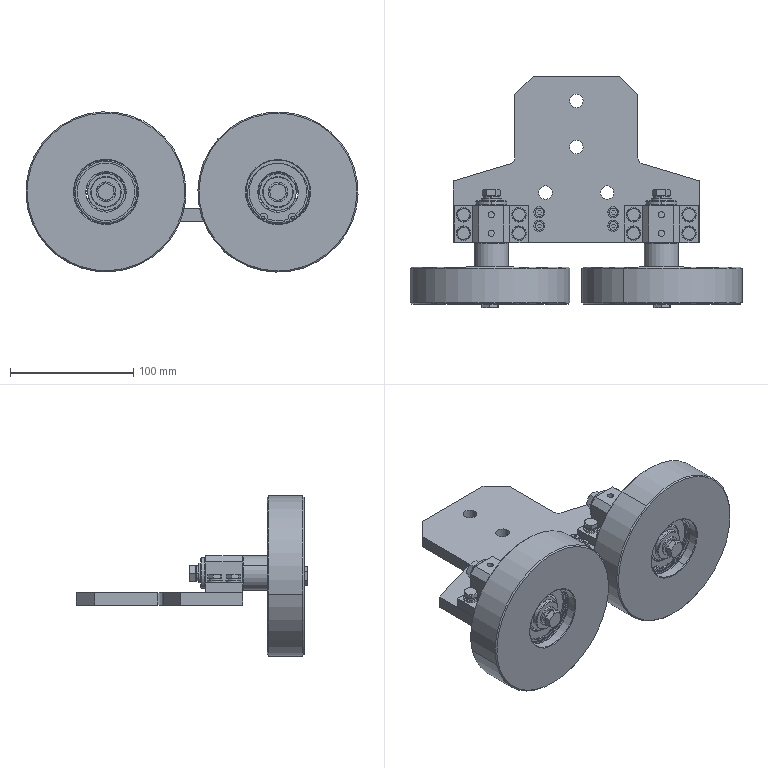Assembly | SolidWorks | mm | 62 component files | 62 solids | 1327 faces | box 269.61 x 188 x 130.18 mm | volume 1018572 mm3 | plane 426 | cylinder 405 | cone 276 | sphere 112 | torus 108 | commonest cylinder face diameters 6 x35 7 x24 6.1 x24 9.282 x24 9 x24 10 x18 4 x16 20 x16
Bill of materials:
Deep Groove Ball Bearing 6304-2RZ | 2 | Alloy Steel | Short annular body made of concentric outer and inner rings. Several spherical elements sit in the annular gap between them, so it looks like a ball-bearing-type body.
Flat Washer C-Class 8×1.6 | 4 | Q235 | Flat circular ring (plain washer shape) with a central through hole and plain flat faces.
Flat Washer C-Class 6×1.6 | 8 | Q235 | Flat circular ring (plain washer shape) with a central through hole. It looks a little thicker compared to its diameter than the other flat rings.
GB_T5781-2000HexHeadBoltFullThreadCGradeM6_20 | 8 | 8.8 Grade | Hex-head bolt shape: a hexagonal head with chamfered corners, a thin washer-face collar underneath, a plain cylindrical shank, and a chamfered tip.
GB_T5781-2000HexHeadBoltFullThreadM8_20 | 4 | 8.8 Grade | Hex-head bolt shape with chamfered head corners, a washer-face collar, a small fillet at the head-to-shank junction, a plain cylindrical shank, and a chamfered end.
GB_T70.1-2000_SocketHeadCapScrew_M4_12 | 4 | 8.8 Grade | Socket-head cap screw shape: a cylindrical head with a hexagonal recess in its top, a plain cylindrical shank, and a chamfered tip.
GB_T93-1987StandardTypeSpringWasher4_1.1 | 4 | 65Mn | Split ring with one radial gap through the full section, similar to a split lock washer. Its rectangular cross-section is fairly thick, and the inner edge appears beveled.
GB_T95-2002FlatWasher4_0.8 | 4 | Steel | Thin, flat circular ring (plain washer shape) with a central through hole. It is thinner compared to its diameter than the other flat rings.
GB893.1-86RetainingRingForHolesTypeA52 | 1 | 65Mn | Thin, open, C-shaped flat ring whose width tapers toward the open ends. Each end has a lug with a small round hole, and the lugs project inward. It resembles an internal retaining ring.
Standard Type Spring Washer (Assembly) 6×1.6 | 8 | 65Mn | Split ring with one radial gap and a rectangular cross-section, similar to a split lock washer. The inner edge appears beveled.
Standard Type Spring Washer (Assembly) 8×2.1 | 4 | 65Mn | Split ring with one radial gap and a rectangular cross-section, similar to a split lock washer. The inner edge appears beveled.
Yk1.5.1AttachmentPlate | 1 | Q235B | Flat plate of constant thickness with a T-like outline: a wide base and a narrower raised tab. The tab has chamfered top corners and filleted inside corners. The plate has a pattern of round through holes.
Yk1.5.2AxisSeat | 2 | 45 | Rectangular base plate with a raised central block centered on it. A large round bore passes horizontally through the block, the block's two upper long edges are chamfered, and the base has four vertical through-holes, two on each side of the block.
Yk1.5.3RollerEccentricAxis | 2 | 45 | Solid stepped round shaft or pin with three coaxial sections: a larger-diameter middle collar, a longer medium-diameter section on one side and a shorter, smaller-diameter section on the other. There is a small axial hole in the end face of the smaller section, and the ends and step edges have small chamfers.
Yk1.5.4NylonRoller | 2 | MC Nylon | Thick flat ring, like a heavy washer or spacer, with a central through-bore that is stepped or counterbored on at least one face. The outer edges have small chamfers.
Yk1.5.5EndCap | 4 | 45 | Thin flat annular disc, like a plain washer, with a central through-hole. The outer edges are chamfered on both faces and the bore edge appears slightly chamfered or rounded.
Mates:
1. coincident | Yk1.5.4NylonRoller-1 face at (98.534, -50, 23.559) dir (0, -1, 0) | Yk1.5.4NylonRoller-2 face at (-41.072, -50, 23.739) dir (0, -1, 0)
2. coincident | Yk1.5.1AttachmentPlate-1 face at (0, 0, 10) dir (0, 0, 1) | Yk1.5.2AxisSeat-1 face at (-10.006, 0, 10) dir (0, 0, -1)
3. coincident | Yk1.5.1AttachmentPlate-1 face at (0, 0, 10) dir (0, 0, 1) | Yk1.5.2AxisSeat-2 face at (67.994, 30, 10) dir (0, 0, -1)
4. distance | Yk1.5.2AxisSeat-1 face at (-40.006, 0, 26) dir (0, 1, 0) r 10 | Yk1.5.2AxisSeat-2 face at (97.994, 30, 26) dir (0, -1, 0) r 10
5. coincident | Yk1.5.1AttachmentPlate-1 face at (128.994, 0, 10) dir (0, -1, 0) | Yk1.5.2AxisSeat-2 face at (97.994, 0, 10) dir (0, -1, 0)
6. concentric | Yk1.5.2AxisSeat-2 face at (120.494, 22.5, 18) dir (0, 0, 1) r 3.5 | GB_T5781-2000HexHeadBoltFullThreadCGradeM6_20-1 face at (120.494, 22.5, 25.2) dir (0, 0, 1) r 3
7. concentric | GB_T5781-2000HexHeadBoltFullThreadCGradeM6_20-1 face at (120.494, 22.5, 25.2) dir (0, 0, 1) r 3 | StandardTypeSpringWasher(Assembly)6_1.6[GB_T93-1987]-1 face at (120.494, 22.5, 21.2) dir (0, 0, -1) r 3.05
8. coincident | GB_T5781-2000HexHeadBoltFullThreadCGradeM6_20-1 face at (130.052, 25.437, 21.2) dir (0, 0, -1) | StandardTypeSpringWasher(Assembly)6_1.6[GB_T93-1987]-1 face at (120.494, 22.5, 21.2) dir (0, 0, 1)
9. concentric | GB_T5781-2000HexHeadBoltFullThreadCGradeM6_20-1 face at (120.494, 22.5, 25.2) dir (0, 0, 1) r 3 | FlatWasherCGrade6_1.6[GB_T95-2002]-1 face at (120.494, 22.5, 9.355) dir (0, 0, -1) r 3.25
10. coincident | StandardTypeSpringWasher(Assembly)6_1.6[GB_T93-1987]-1 face at (120.494, 22.5, 19.6) dir (0, 0, -1) | FlatWasherCGrade6_1.6[GB_T95-2002]-1 face at (117.244, 22.5, 19.6) dir (0, 0, 1)
11. coincident | Yk1.5.2AxisSeat-2 face at (127.994, 30, 18) dir (0, 0, 1) | FlatWasherCGrade6_1.6[GB_T95-2002]-1 face at (117.244, 22.5, 18) dir (0, 0, -1)
12. concentric | Yk1.5.4NylonRoller-1 face at (98.534, -25, 23.559) dir (0, -1, 0) r 26 | DeepGrooveBallBearing6304-2RZ[GB_T276-94]-1 face at (98.534, -20.079, 23.559) dir (0, 1, 0) r 10
13. coincident | Yk1.5.4NylonRoller-1 face at (98.534, -25, 23.559) dir (0, -1, 0) | DeepGrooveBallBearing6304-2RZ[GB_T276-94]-1 face at (86.06, -25, 15.41) dir (0, 1, 0)
14. coincident | Yk1.5.2AxisSeat-1 face at (-40.006, 30, 10) dir (0, 1, 0) | Yk1.5.2AxisSeat-2 face at (97.994, 30, 10) dir (0, 1, 0)
15. width | Yk1.5.2AxisSeat-1 face at (-70.006, 0, 10) dir (-1, 0, 0) | Yk1.5.2AxisSeat-2 face at (127.994, 30, 10) dir (1, 0, 0) | Yk1.5.1AttachmentPlate-1 face at (128.994, 50, 10) dir (1, 0, 0) | Yk1.5.1AttachmentPlate-1 face at (-71.006, 0, 10) dir (-1, 0, 0)
16. concentric | Yk1.5.4NylonRoller-2 face at (-41.072, -50, 23.739) dir (0, 1, 0) r 19 | DeepGrooveBallBearing6304-2RZ[GB_T276-94]-2 face at (-41.072, -20.079, 23.739) dir (0, 1, 0) r 10
17. coincident | Yk1.5.4NylonRoller-2 face at (-41.072, -25, 23.739) dir (0, -1, 0) | DeepGrooveBallBearing6304-2RZ[GB_T276-94]-2 face at (-53.546, -25, 15.589) dir (0, 1, 0)
18. concentric | Yk1.5.2AxisSeat-1 face at (-40.006, 0, 26) dir (0, 1, 0) r 10 | Yk1.5.5EndCap-1 face at (-40.006, 34, 26) dir (0, -1, 0) r 4.5
19. coincident | Yk1.5.2AxisSeat-1 face at (-40.006, 30, 10) dir (0, 1, 0) | Yk1.5.5EndCap-1 face at (-40.006, 30, 26) dir (0, -1, 0)
20. concentric | DeepGrooveBallBearing6304-2RZ[GB_T276-94]-1 face at (98.534, -20.079, 23.559) dir (0, 1, 0) r 10 | Yk1.5.3RollerEccentricAxis-2 face at (98.534, -40, 23.559) dir (0, 1, 0) r 10
21. concentric | DeepGrooveBallBearing6304-2RZ[GB_T276-94]-2 face at (-41.072, -20.079, 23.739) dir (0, 1, 0) r 10 | Yk1.5.3RollerEccentricAxis-1 face at (-41.072, -40, 23.739) dir (0, 1, 0) r 10
22. concentric | Yk1.5.2AxisSeat-1 face at (-40.006, 0, 26) dir (0, 1, 0) r 10 | Yk1.5.3RollerEccentricAxis-1 face at (-40.006, -57.214, 26) dir (0, -1, 0) r 10
23. coincident | DeepGrooveBallBearing6304-2RZ[GB_T276-94]-2 face at (-53.546, -25, 15.589) dir (0, 1, 0) | Yk1.5.3RollerEccentricAxis-1 face at (-45.974, -25, 13.336) dir (0, -1, 0)
24. coincident | Yk1.5.2AxisSeat-1 face at (-40.006, 0, 10) dir (0, -1, 0) | Yk1.5.3RollerEccentricAxis-1 face at (-44.269, 0, 16.954) dir (0, 1, 0)
25. concentric | Yk1.5.2AxisSeat-2 face at (97.994, 30, 26) dir (0, -1, 0) r 10 | Yk1.5.3RollerEccentricAxis-2 face at (97.994, -57.214, 26) dir (0, -1, 0) r 10
26. concentric | Yk1.5.4NylonRoller-1 face at (98.534, -25, 23.559) dir (0, -1, 0) r 26 | Yk1.5.3RollerEccentricAxis-2 face at (98.534, -40, 23.559) dir (0, 1, 0) r 10
27. coincident | Yk1.5.2AxisSeat-2 face at (97.994, 0, 10) dir (0, -1, 0) | Yk1.5.3RollerEccentricAxis-2 face at (100.154, 0, 16.236) dir (0, 1, 0)
28. concentric | Yk1.5.4NylonRoller-1 face at (98.534, -25, 23.559) dir (0, -1, 0) r 26 | GB893.1-86RetainingRingForHolesTypeA52-1 face at (98.534, -42, 23.559) dir (0, 1, 0) r 27.5
29. coincident | Yk1.5.4NylonRoller-1 face at (98.534, -40, 23.559) dir (0, -1, 0) | GB893.1-86RetainingRingForHolesTypeA52-1 face at (86.978, -40, 3.5) dir (0, 1, 0)
30. concentric | StandardTypeSpringWasher(Assembly)8_2.1[GB_T93-1987]-1 face at (-40.006, 35.6, 26) dir (0, 1, 0) r 4.05 | FlatWasherC-Class8_1.6[GB_T95-2002]-1 face at (-40.006, 25.355, 26) dir (0, -1, 0) r 4.5
31. coincident | StandardTypeSpringWasher(Assembly)8_2.1[GB_T93-1987]-1 face at (-40.006, 35.6, 26) dir (0, -1, 0) | FlatWasherC-Class8_1.6[GB_T95-2002]-1 face at (-44.506, 35.6, 26) dir (0, 1, 0)
32. coincident | Yk1.5.5EndCap-1 face at (-40.006, 34, 26) dir (0, 1, 0) | FlatWasherC-Class8_1.6[GB_T95-2002]-1 face at (-44.506, 34, 26) dir (0, -1, 0)
33. concentric | Yk1.5.5EndCap-1 face at (-40.006, 34, 26) dir (0, -1, 0) r 4.5 | StandardTypeSpringWasher(Assembly)8_2.1[GB_T93-1987]-1 face at (-40.006, 35.6, 26) dir (0, 1, 0) r 4.05
34. concentric | Yk1.5.5EndCap-1 face at (-40.006, 34, 26) dir (0, -1, 0) r 4.5 | GB_T5781-2000HexHeadBoltFullThreadM8_20-1 face at (-40.006, 43, 26) dir (0, 1, 0) r 4
35. coincident | StandardTypeSpringWasher(Assembly)8_2.1[GB_T93-1987]-1 face at (-40.006, 37.7, 26) dir (0, 1, 0) | GB_T5781-2000HexHeadBoltFullThreadM8_20-1 face at (-32.501, 37.7, 26) dir (0, -1, 0)
36. coincident | DeepGrooveBallBearing6304-2RZ[GB_T276-94]-2 face at (-53.546, -40, 15.589) dir (0, -1, 0) | Yk1.5.5EndCap-4 face at (-41.072, -40, 23.739) dir (0, 1, 0)
37. concentric | Yk1.5.3RollerEccentricAxis-1 face at (-41.072, -40, 23.739) dir (0, -1, 0) r 4 | Yk1.5.5EndCap-4 face at (-41.072, -40, 23.739) dir (0, -1, 0) r 4.5
38. concentric | FlatWasherC-Class8_1.6[GB_T95-2002]-2 face at (-41.072, -54.245, 23.739) dir (0, -1, 0) r 4.5 | StandardTypeSpringWasher(Assembly)8_2.1[GB_T93-1987]-2 face at (-41.072, -47.7, 23.739) dir (0, 1, 0) r 4.05
39. coincident | FlatWasherC-Class8_1.6[GB_T95-2002]-2 face at (-45.572, -45.6, 23.739) dir (0, -1, 0) | StandardTypeSpringWasher(Assembly)8_2.1[GB_T93-1987]-2 face at (-41.072, -45.6, 23.739) dir (0, 1, 0)
40. concentric | StandardTypeSpringWasher(Assembly)8_2.1[GB_T93-1987]-2 face at (-41.072, -47.7, 23.739) dir (0, 1, 0) r 4.05 | GB_T5781-2000HexHeadBoltFullThreadM8_20-2 face at (-41.072, -53, 23.739) dir (0, -1, 0) r 4
41. coincident | StandardTypeSpringWasher(Assembly)8_2.1[GB_T93-1987]-2 face at (-41.072, -47.7, 23.739) dir (0, -1, 0) | GB_T5781-2000HexHeadBoltFullThreadM8_20-2 face at (-47.356, -47.7, 19.633) dir (0, 1, 0)
42. coincident | Yk1.5.5EndCap-4 face at (-41.072, -44, 23.739) dir (0, -1, 0) | FlatWasherC-Class8_1.6[GB_T95-2002]-2 face at (-45.572, -44, 23.739) dir (0, 1, 0)
43. concentric | Yk1.5.5EndCap-4 face at (-41.072, -40, 23.739) dir (0, -1, 0) r 4.5 | GB_T5781-2000HexHeadBoltFullThreadM8_20-2 face at (-41.072, -53, 23.739) dir (0, -1, 0) r 4
44. concentric | Yk1.5.5EndCap-5 face at (98.534, -40, 23.559) dir (0, -1, 0) r 4.5 | FlatWasherC-Class8_1.6[GB_T95-2002]-3 face at (98.534, -54.245, 23.559) dir (0, -1, 0) r 4.5
45. concentric | Yk1.5.5EndCap-5 face at (98.534, -40, 23.559) dir (0, -1, 0) r 4.5 | FlatWasherC-Class8_1.6[GB_T95-2002]-3 face at (98.534, -54.245, 23.559) dir (0, -1, 0) r 4.5
46. concentric | FlatWasherC-Class8_1.6[GB_T95-2002]-3 face at (98.534, -54.245, 23.559) dir (0, -1, 0) r 4.5 | StandardTypeSpringWasher(Assembly)8_2.1[GB_T93-1987]-3 face at (98.534, -47.7, 23.559) dir (0, 1, 0) r 4.05
47. coincident | Yk1.5.5EndCap-5 face at (98.534, -44, 23.559) dir (0, -1, 0) | FlatWasherC-Class8_1.6[GB_T95-2002]-3 face at (94.034, -44, 23.559) dir (0, 1, 0)
48. coincident | FlatWasherC-Class8_1.6[GB_T95-2002]-3 face at (94.034, -45.6, 23.559) dir (0, -1, 0) | StandardTypeSpringWasher(Assembly)8_2.1[GB_T93-1987]-3 face at (98.534, -45.6, 23.559) dir (0, 1, 0)
49. concentric | StandardTypeSpringWasher(Assembly)8_2.1[GB_T93-1987]-3 face at (98.534, -47.7, 23.559) dir (0, 1, 0) r 4.05 | GB_T5781-2000HexHeadBoltFullThreadM8_20-3 face at (98.534, -53, 23.559) dir (0, -1, 0) r 4
50. coincident | StandardTypeSpringWasher(Assembly)8_2.1[GB_T93-1987]-3 face at (98.534, -47.7, 23.559) dir (0, -1, 0) | GB_T5781-2000HexHeadBoltFullThreadM8_20-3 face at (92.25, -47.7, 19.454) dir (0, 1, 0)
51. coincident | Yk1.5.3RollerEccentricAxis-2 face at (98.534, -40, 23.559) dir (0, -1, 0) | Yk1.5.5EndCap-5 face at (98.534, -40, 23.559) dir (0, 1, 0)
52. concentric | Yk1.5.3RollerEccentricAxis-2 face at (98.534, -40, 23.559) dir (0, -1, 0) r 4 | Yk1.5.5EndCap-5 face at (98.534, -40, 23.559) dir (0, -1, 0) r 12.5
53. concentric | Yk1.5.5EndCap-6 face at (97.994, 34, 26) dir (0, -1, 0) r 4.5 | FlatWasherC-Class8_1.6[GB_T95-2002]-4 face at (97.994, 25.355, 26) dir (0, -1, 0) r 4.5
54. concentric | Yk1.5.5EndCap-6 face at (97.994, 34, 26) dir (0, -1, 0) r 4.5 | StandardTypeSpringWasher(Assembly)8_2.1[GB_T93-1987]-4 face at (97.994, 35.6, 26) dir (0, 1, 0) r 4.05
55. concentric | StandardTypeSpringWasher(Assembly)8_2.1[GB_T93-1987]-4 face at (97.994, 35.6, 26) dir (0, 1, 0) r 4.05 | GB_T5781-2000HexHeadBoltFullThreadM8_20-4 face at (97.994, 43, 26) dir (0, 1, 0) r 4
56. coincident | Yk1.5.5EndCap-6 face at (97.994, 34, 26) dir (0, 1, 0) | FlatWasherC-Class8_1.6[GB_T95-2002]-4 face at (93.494, 34, 26) dir (0, -1, 0)
57. coincident | FlatWasherC-Class8_1.6[GB_T95-2002]-4 face at (93.494, 35.6, 26) dir (0, 1, 0) | StandardTypeSpringWasher(Assembly)8_2.1[GB_T93-1987]-4 face at (97.994, 35.6, 26) dir (0, -1, 0)
58. coincident | StandardTypeSpringWasher(Assembly)8_2.1[GB_T93-1987]-4 face at (97.994, 37.7, 26) dir (0, 1, 0) | GB_T5781-2000HexHeadBoltFullThreadM8_20-4 face at (105.499, 37.7, 26) dir (0, -1, 0)
59. coincident | Yk1.5.2AxisSeat-2 face at (97.994, 30, 10) dir (0, 1, 0) | Yk1.5.5EndCap-6 face at (97.994, 30, 26) dir (0, -1, 0)
60. concentric | Yk1.5.3RollerEccentricAxis-2 face at (97.994, 29, 26) dir (0, 1, 0) r 4 | Yk1.5.5EndCap-6 face at (97.994, 34, 26) dir (0, -1, 0) r 12.5
61. concentric | GB_T95-2002FlatWasher4_0.8-1 face at (-1.006, 24.5, 3.355) dir (0, 0, -1) r 2.25 | GB_T93-1987StandardTypeSpringWasher4_1.1-1 face at (-1.006, 24.5, 12.8) dir (0, 0, 1) r 2.05
62. coincident | GB_T95-2002FlatWasher4_0.8-1 face at (-3.256, 24.5, 12.8) dir (0, 0, 1) | GB_T93-1987StandardTypeSpringWasher4_1.1-1 face at (-1.006, 24.5, 12.8) dir (0, 0, -1)
63. coincident | GB_T93-1987StandardTypeSpringWasher4_1.1-1 face at (-1.006, 24.5, 13.9) dir (0, 0, 1) | GB_T70.1-2000_SocketHeadCapScrew_M4_12-1 face at (-1.006, 28, 13.9) dir (0, 0, -1)